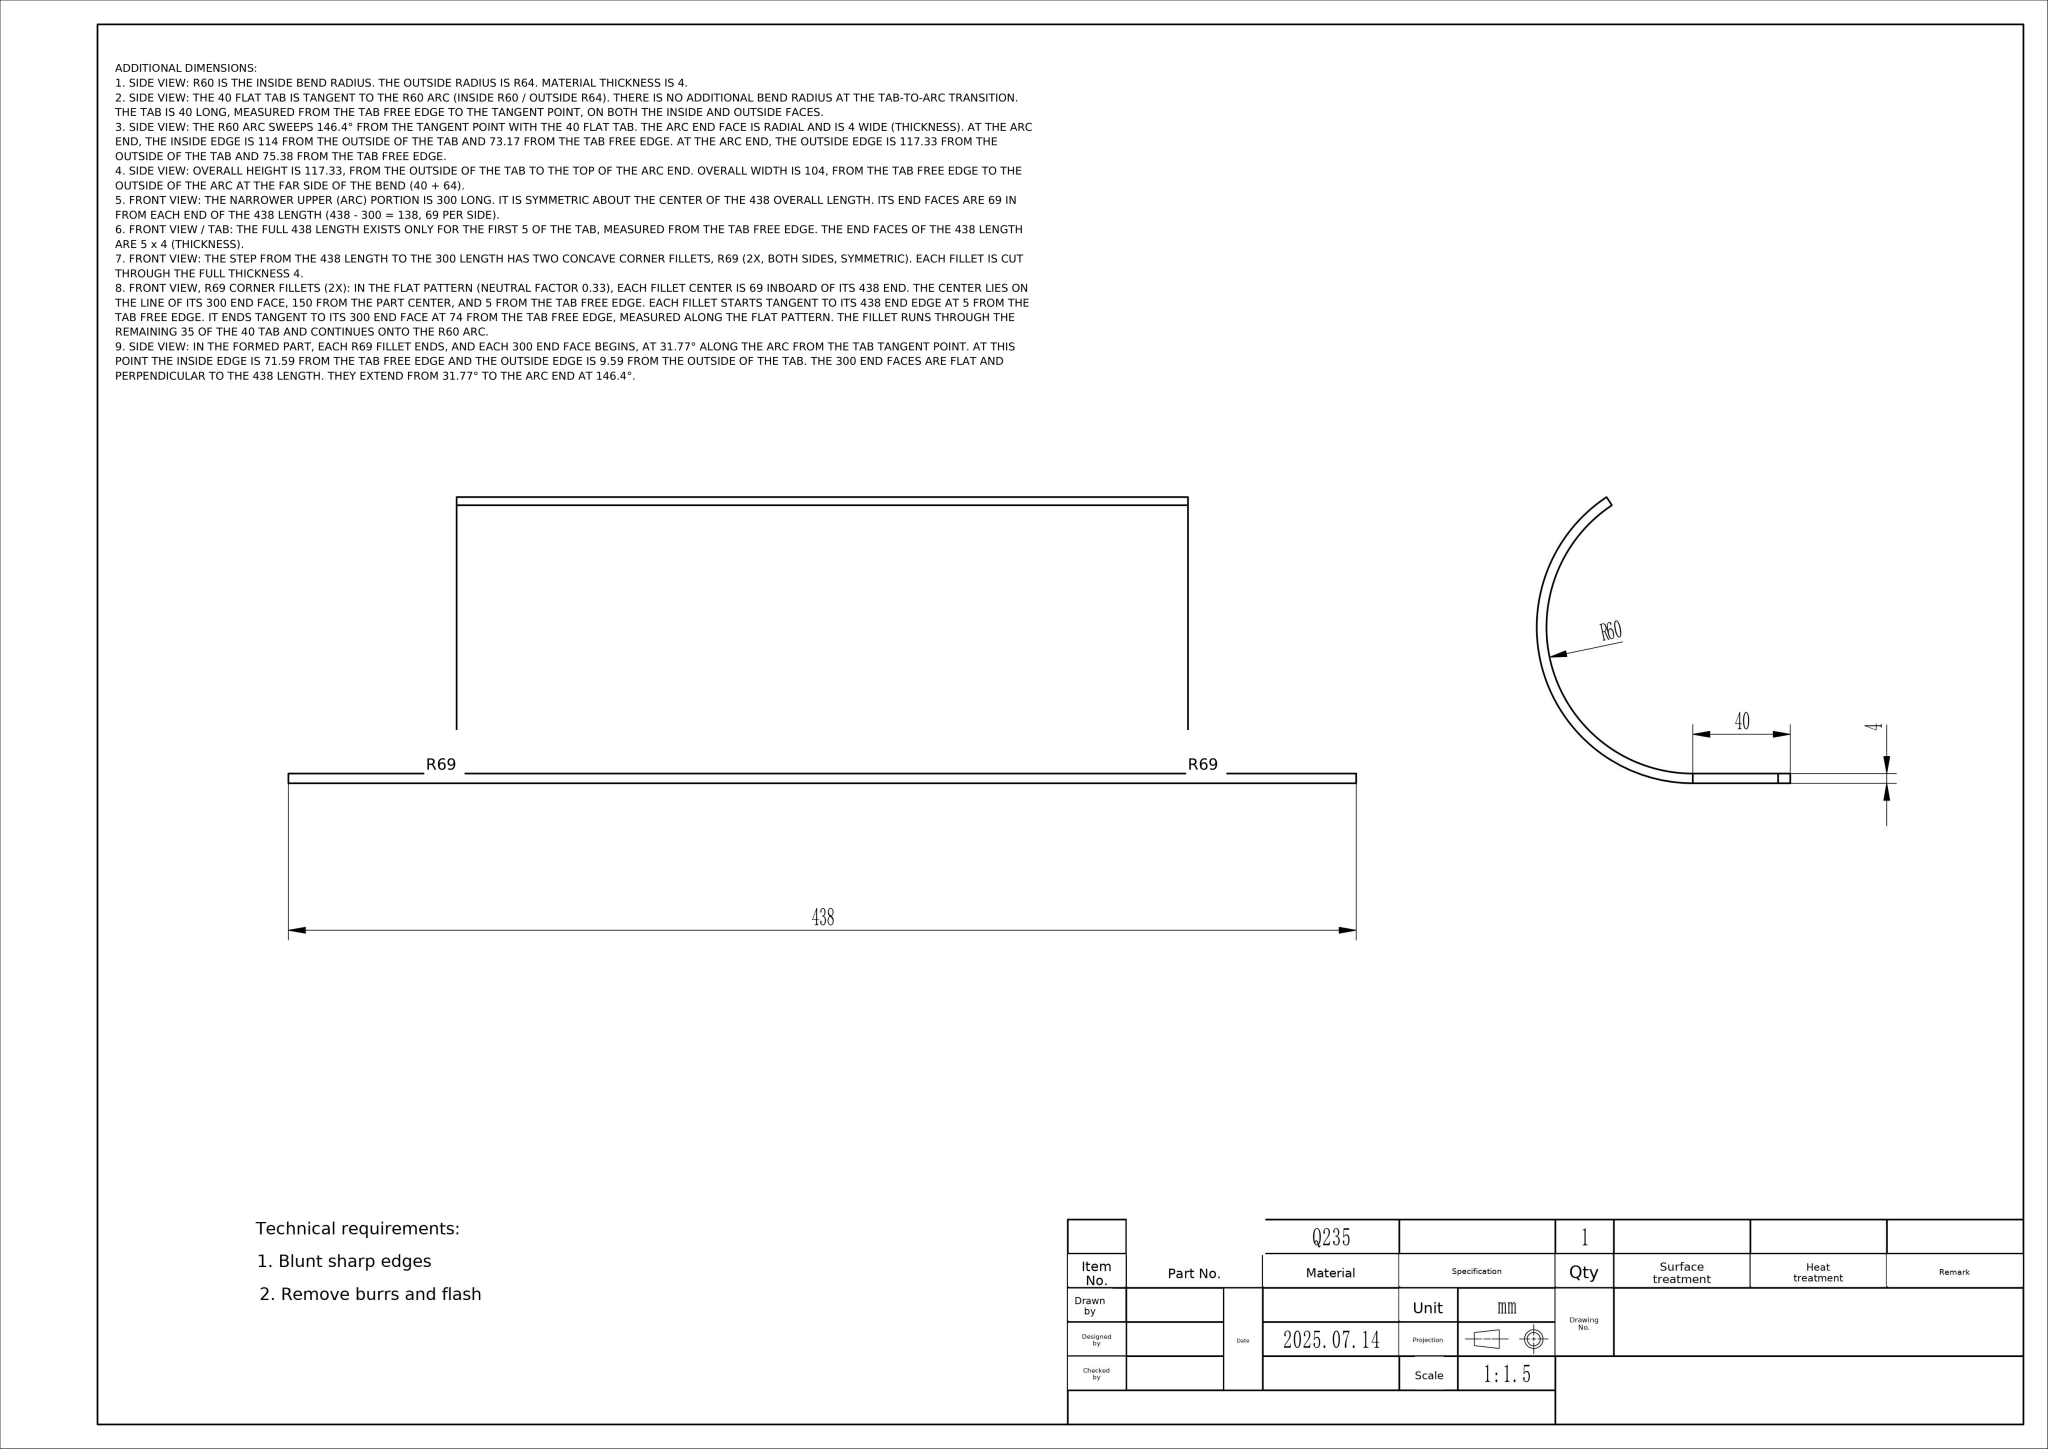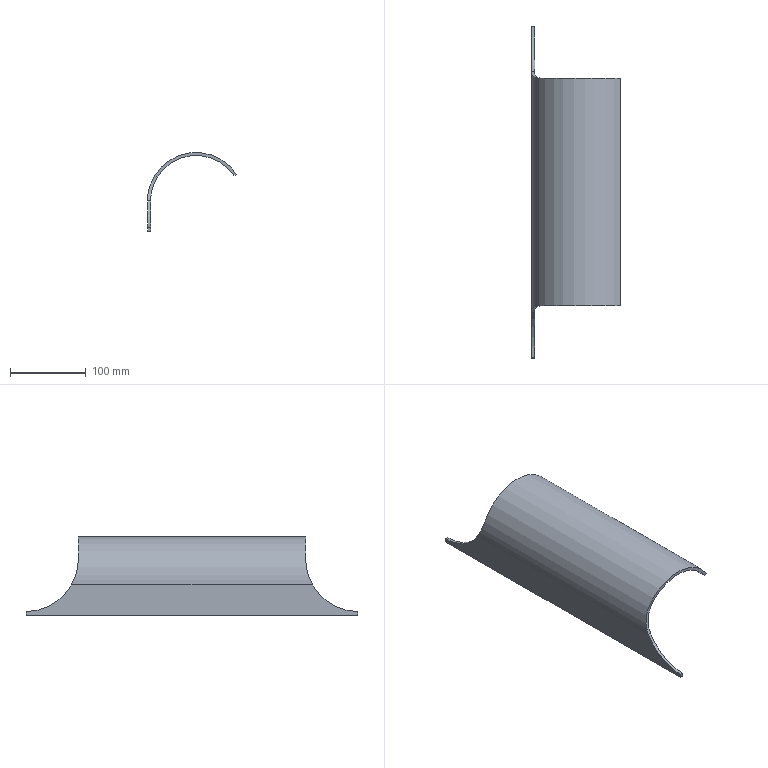Part | NX | mm | 1 solid | 14 faces | box 117.33 x 438 x 104 mm | volume 249102 mm3 | plane 8 | cylinder 4 | spline 2 | commonest cylinder face diameters 138 x2 128 x1 120 x1
STEP:
#1=CARTESIAN_POINT('',(0.,0.,0.));
#2=DIRECTION('',(0.,0.,1.));
#3=DIRECTION('',(1.,0.,0.));
#4=AXIS2_PLACEMENT_3D('',#1,#2,#3);
#5=(LENGTH_UNIT()NAMED_UNIT(*)SI_UNIT(.MILLI.,.METRE.));
#6=UNCERTAINTY_MEASURE_WITH_UNIT(LENGTH_MEASURE(0.0508),#5,'','');
#7=(NAMED_UNIT(*)PLANE_ANGLE_UNIT()SI_UNIT($,.RADIAN.));
#8=PLANE_ANGLE_MEASURE_WITH_UNIT(PLANE_ANGLE_MEASURE(0.01745),#7);
#9=DIMENSIONAL_EXPONENTS(0.,0.,0.,0.,0.,0.,0.);
#10=(CONVERSION_BASED_UNIT('',#8)NAMED_UNIT(#9)PLANE_ANGLE_UNIT());
#11=(NAMED_UNIT(*)SI_UNIT($,.STERADIAN.)SOLID_ANGLE_UNIT());
#12=(GEOMETRIC_REPRESENTATION_CONTEXT(3)GLOBAL_UNCERTAINTY_ASSIGNED_CONTEXT((#6))GLOBAL_UNIT_ASSIGNED_CONTEXT((#5,#10,#11))REPRESENTATION_CONTEXT('',''));
#13=SHAPE_REPRESENTATION('',(#4),#12);
#14=CARTESIAN_POINT('',(-0.,-158.958,40.));
#15=VERTEX_POINT('',#14);
#16=CARTESIAN_POINT('',(0.,-219.,5.));
#17=VERTEX_POINT('',#16);
#18=CARTESIAN_POINT('',(0.,-219.,74.));
#19=DIRECTION('',(-1.,0.,0.));
#20=DIRECTION('',(0.,1.,0.));
#21=AXIS2_PLACEMENT_3D('',#18,#19,#20);
#22=CIRCLE('',#21,69.);
#23=EDGE_CURVE('',#15,#17,#22,.T.);
#24=ORIENTED_EDGE('',*,*,#23,.F.);
#25=CARTESIAN_POINT('',(-4.,-158.958,40.));
#26=VERTEX_POINT('',#25);
#27=CARTESIAN_POINT('',(-4.,-158.958,40.));
#28=DIRECTION('',(-1.,0.,0.));
#29=VECTOR('',#28,1.);
#30=LINE('',#27,#29);
#31=EDGE_CURVE('',#15,#26,#30,.T.);
#32=ORIENTED_EDGE('',*,*,#31,.T.);
#33=CARTESIAN_POINT('',(-4.,-219.,5.));
#34=VERTEX_POINT('',#33);
#35=CARTESIAN_POINT('',(-4.,-219.,74.));
#36=DIRECTION('',(-1.,0.,0.));
#37=DIRECTION('',(0.,1.,0.));
#38=AXIS2_PLACEMENT_3D('',#35,#36,#37);
#39=CIRCLE('',#38,69.);
#40=EDGE_CURVE('',#26,#34,#39,.T.);
#41=ORIENTED_EDGE('',*,*,#40,.T.);
#42=CARTESIAN_POINT('',(-4.,-219.,5.));
#43=DIRECTION('',(-1.,0.,0.));
#44=VECTOR('',#43,1.);
#45=LINE('',#42,#44);
#46=EDGE_CURVE('',#17,#34,#45,.T.);
#47=ORIENTED_EDGE('',*,*,#46,.F.);
#48=EDGE_LOOP('',(#24,#32,#41,#47));
#49=FACE_OUTER_BOUND('',#48,.T.);
#50=CARTESIAN_POINT('',(-4.,-219.,74.));
#51=DIRECTION('',(1.,0.,-0.));
#52=DIRECTION('',(0.,0.,-1.));
#53=AXIS2_PLACEMENT_3D('',#50,#51,#52);
#54=CYLINDRICAL_SURFACE('',#53,69.);
#55=ADVANCED_FACE('',(#49),#54,.F.);
#56=CARTESIAN_POINT('',(0.,219.,0.));
#57=VERTEX_POINT('',#56);
#58=CARTESIAN_POINT('',(0.,-219.,-0.));
#59=VERTEX_POINT('',#58);
#60=CARTESIAN_POINT('',(0.,-150.,0.));
#61=DIRECTION('',(0.,-1.,0.));
#62=VECTOR('',#61,1.);
#63=LINE('',#60,#62);
#64=EDGE_CURVE('',#57,#59,#63,.T.);
#65=ORIENTED_EDGE('',*,*,#64,.T.);
#66=CARTESIAN_POINT('',(-4.,-219.,-0.));
#67=VERTEX_POINT('',#66);
#68=CARTESIAN_POINT('',(-4.,-219.,-0.));
#69=DIRECTION('',(-1.,0.,0.));
#70=VECTOR('',#69,1.);
#71=LINE('',#68,#70);
#72=EDGE_CURVE('',#59,#67,#71,.T.);
#73=ORIENTED_EDGE('',*,*,#72,.T.);
#74=CARTESIAN_POINT('',(-4.,219.,0.));
#75=VERTEX_POINT('',#74);
#76=CARTESIAN_POINT('',(-4.,-150.,0.));
#77=DIRECTION('',(0.,-1.,0.));
#78=VECTOR('',#77,1.);
#79=LINE('',#76,#78);
#80=EDGE_CURVE('',#75,#67,#79,.T.);
#81=ORIENTED_EDGE('',*,*,#80,.F.);
#82=CARTESIAN_POINT('',(-4.,219.,0.));
#83=DIRECTION('',(-1.,0.,0.));
#84=VECTOR('',#83,1.);
#85=LINE('',#82,#84);
#86=EDGE_CURVE('',#57,#75,#85,.T.);
#87=ORIENTED_EDGE('',*,*,#86,.F.);
#88=EDGE_LOOP('',(#65,#73,#81,#87));
#89=FACE_OUTER_BOUND('',#88,.T.);
#90=CARTESIAN_POINT('',(0.,-150.,0.));
#91=DIRECTION('',(0.,0.,1.));
#92=DIRECTION('',(0.,1.,0.));
#93=AXIS2_PLACEMENT_3D('',#90,#91,#92);
#94=PLANE('',#93);
#95=ADVANCED_FACE('',(#89),#94,.F.);
#96=CARTESIAN_POINT('',(-4.,158.958,40.));
#97=VERTEX_POINT('',#96);
#98=CARTESIAN_POINT('',(-4.,-150.,40.));
#99=DIRECTION('',(0.,-1.,0.));
#100=VECTOR('',#99,1.);
#101=LINE('',#98,#100);
#102=EDGE_CURVE('',#97,#26,#101,.T.);
#103=ORIENTED_EDGE('',*,*,#102,.F.);
#104=CARTESIAN_POINT('',(-4.,219.,5.));
#105=VERTEX_POINT('',#104);
#106=CARTESIAN_POINT('',(-4.,219.,74.));
#107=DIRECTION('',(1.,0.,0.));
#108=DIRECTION('',(0.,1.,0.));
#109=AXIS2_PLACEMENT_3D('',#106,#107,#108);
#110=CIRCLE('',#109,69.);
#111=EDGE_CURVE('',#97,#105,#110,.T.);
#112=ORIENTED_EDGE('',*,*,#111,.T.);
#113=CARTESIAN_POINT('',(-4.,219.,0.));
#114=DIRECTION('',(0.,0.,-1.));
#115=VECTOR('',#114,1.);
#116=LINE('',#113,#115);
#117=EDGE_CURVE('',#105,#75,#116,.T.);
#118=ORIENTED_EDGE('',*,*,#117,.T.);
#119=ORIENTED_EDGE('',*,*,#80,.T.);
#120=CARTESIAN_POINT('',(-4.,-219.,-0.));
#121=DIRECTION('',(0.,0.,-1.));
#122=VECTOR('',#121,1.);
#123=LINE('',#120,#122);
#124=EDGE_CURVE('',#34,#67,#123,.T.);
#125=ORIENTED_EDGE('',*,*,#124,.F.);
#126=ORIENTED_EDGE('',*,*,#40,.F.);
#127=EDGE_LOOP('',(#103,#112,#118,#119,#125,#126));
#128=FACE_OUTER_BOUND('',#127,.T.);
#129=CARTESIAN_POINT('',(-4.,-150.,0.));
#130=DIRECTION('',(-1.,0.,0.));
#131=DIRECTION('',(0.,0.,1.));
#132=AXIS2_PLACEMENT_3D('',#129,#130,#131);
#133=PLANE('',#132);
#134=ADVANCED_FACE('',(#128),#133,.T.);
#135=ORIENTED_EDGE('',*,*,#64,.F.);
#136=CARTESIAN_POINT('',(0.,219.,5.));
#137=VERTEX_POINT('',#136);
#138=CARTESIAN_POINT('',(0.,219.,0.));
#139=DIRECTION('',(0.,0.,-1.));
#140=VECTOR('',#139,1.);
#141=LINE('',#138,#140);
#142=EDGE_CURVE('',#137,#57,#141,.T.);
#143=ORIENTED_EDGE('',*,*,#142,.F.);
#144=CARTESIAN_POINT('',(0.,158.958,40.));
#145=VERTEX_POINT('',#144);
#146=CARTESIAN_POINT('',(0.,219.,74.));
#147=DIRECTION('',(1.,0.,0.));
#148=DIRECTION('',(0.,1.,0.));
#149=AXIS2_PLACEMENT_3D('',#146,#147,#148);
#150=CIRCLE('',#149,69.);
#151=EDGE_CURVE('',#145,#137,#150,.T.);
#152=ORIENTED_EDGE('',*,*,#151,.F.);
#153=CARTESIAN_POINT('',(0.,-150.,40.));
#154=DIRECTION('',(0.,-1.,0.));
#155=VECTOR('',#154,1.);
#156=LINE('',#153,#155);
#157=EDGE_CURVE('',#145,#15,#156,.T.);
#158=ORIENTED_EDGE('',*,*,#157,.T.);
#159=ORIENTED_EDGE('',*,*,#23,.T.);
#160=CARTESIAN_POINT('',(0.,-219.,-0.));
#161=DIRECTION('',(0.,0.,-1.));
#162=VECTOR('',#161,1.);
#163=LINE('',#160,#162);
#164=EDGE_CURVE('',#17,#59,#163,.T.);
#165=ORIENTED_EDGE('',*,*,#164,.T.);
#166=EDGE_LOOP('',(#135,#143,#152,#158,#159,#165));
#167=FACE_OUTER_BOUND('',#166,.T.);
#168=CARTESIAN_POINT('',(0.,-150.,0.));
#169=DIRECTION('',(-1.,0.,0.));
#170=DIRECTION('',(0.,0.,1.));
#171=AXIS2_PLACEMENT_3D('',#168,#169,#170);
#172=PLANE('',#171);
#173=ADVANCED_FACE('',(#167),#172,.F.);
#174=ORIENTED_EDGE('',*,*,#142,.T.);
#175=ORIENTED_EDGE('',*,*,#86,.T.);
#176=ORIENTED_EDGE('',*,*,#117,.F.);
#177=CARTESIAN_POINT('',(-4.,219.,5.));
#178=DIRECTION('',(-1.,0.,0.));
#179=VECTOR('',#178,1.);
#180=LINE('',#177,#179);
#181=EDGE_CURVE('',#137,#105,#180,.T.);
#182=ORIENTED_EDGE('',*,*,#181,.F.);
#183=EDGE_LOOP('',(#174,#175,#176,#182));
#184=FACE_OUTER_BOUND('',#183,.T.);
#185=CARTESIAN_POINT('',(-4.,219.,0.));
#186=DIRECTION('',(0.,1.,0.));
#187=DIRECTION('',(0.,0.,1.));
#188=AXIS2_PLACEMENT_3D('',#185,#186,#187);
#189=PLANE('',#188);
#190=ADVANCED_FACE('',(#184),#189,.T.);
#191=CARTESIAN_POINT('',(-4.,158.958,40.));
#192=DIRECTION('',(-1.,0.,0.));
#193=VECTOR('',#192,1.);
#194=LINE('',#191,#193);
#195=EDGE_CURVE('',#145,#97,#194,.T.);
#196=ORIENTED_EDGE('',*,*,#195,.F.);
#197=ORIENTED_EDGE('',*,*,#151,.T.);
#198=ORIENTED_EDGE('',*,*,#181,.T.);
#199=ORIENTED_EDGE('',*,*,#111,.F.);
#200=EDGE_LOOP('',(#196,#197,#198,#199));
#201=FACE_OUTER_BOUND('',#200,.T.);
#202=CARTESIAN_POINT('',(-4.,219.,74.));
#203=DIRECTION('',(1.,0.,-0.));
#204=DIRECTION('',(0.,0.,-1.));
#205=AXIS2_PLACEMENT_3D('',#202,#203,#204);
#206=CYLINDRICAL_SURFACE('',#205,69.);
#207=ADVANCED_FACE('',(#201),#206,.F.);
#208=ORIENTED_EDGE('',*,*,#164,.F.);
#209=ORIENTED_EDGE('',*,*,#46,.T.);
#210=ORIENTED_EDGE('',*,*,#124,.T.);
#211=ORIENTED_EDGE('',*,*,#72,.F.);
#212=EDGE_LOOP('',(#208,#209,#210,#211));
#213=FACE_OUTER_BOUND('',#212,.T.);
#214=CARTESIAN_POINT('',(-4.,-219.,-0.));
#215=DIRECTION('',(0.,1.,0.));
#216=DIRECTION('',(0.,0.,1.));
#217=AXIS2_PLACEMENT_3D('',#214,#215,#216);
#218=PLANE('',#217);
#219=ADVANCED_FACE('',(#213),#218,.F.);
#220=CARTESIAN_POINT('',(110.,150.,73.166));
#221=VERTEX_POINT('',#220);
#222=CARTESIAN_POINT('',(113.333,150.,75.377));
#223=VERTEX_POINT('',#222);
#224=CARTESIAN_POINT('',(113.333,150.,75.377));
#225=DIRECTION('',(0.8333,0.,0.5528));
#226=VECTOR('',#225,1.);
#227=LINE('',#224,#226);
#228=EDGE_CURVE('',#221,#223,#227,.T.);
#229=ORIENTED_EDGE('',*,*,#228,.F.);
#230=CARTESIAN_POINT('',(8.989,150.,71.589));
#231=VERTEX_POINT('',#230);
#232=CARTESIAN_POINT('',(60.,150.,40.));
#233=DIRECTION('',(-0.,-1.,-0.));
#234=DIRECTION('',(0.,0.,1.));
#235=AXIS2_PLACEMENT_3D('',#232,#233,#234);
#236=CIRCLE('',#235,60.);
#237=EDGE_CURVE('',#221,#231,#236,.T.);
#238=ORIENTED_EDGE('',*,*,#237,.T.);
#239=CARTESIAN_POINT('',(5.588,150.,73.695));
#240=VERTEX_POINT('',#239);
#241=CARTESIAN_POINT('',(8.989,150.,71.589));
#242=DIRECTION('',(0.8502,0.,-0.5265));
#243=VECTOR('',#242,1.);
#244=LINE('',#241,#243);
#245=EDGE_CURVE('',#240,#231,#244,.T.);
#246=ORIENTED_EDGE('',*,*,#245,.F.);
#247=CARTESIAN_POINT('',(60.,150.,40.));
#248=DIRECTION('',(-0.,-1.,-0.));
#249=DIRECTION('',(1.,0.,0.));
#250=AXIS2_PLACEMENT_3D('',#247,#248,#249);
#251=CIRCLE('',#250,64.);
#252=EDGE_CURVE('',#223,#240,#251,.T.);
#253=ORIENTED_EDGE('',*,*,#252,.F.);
#254=EDGE_LOOP('',(#229,#238,#246,#253));
#255=FACE_OUTER_BOUND('',#254,.T.);
#256=CARTESIAN_POINT('',(60.,150.,40.));
#257=DIRECTION('',(0.,1.,0.));
#258=DIRECTION('',(0.,-0.,1.));
#259=AXIS2_PLACEMENT_3D('',#256,#257,#258);
#260=PLANE('',#259);
#261=ADVANCED_FACE('',(#255),#260,.T.);
#262=ORIENTED_EDGE('',*,*,#245,.T.);
#263=CARTESIAN_POINT('',(8.989,150.,71.589));
#264=CARTESIAN_POINT('',(7.463,150.,69.125));
#265=CARTESIAN_POINT('',(6.117,150.191,66.549));
#266=CARTESIAN_POINT('',(3.825,150.952,61.276));
#267=CARTESIAN_POINT('',(2.88,151.522,58.578));
#268=CARTESIAN_POINT('',(1.397,153.032,53.172));
#269=CARTESIAN_POINT('',(0.8583,153.972,50.463));
#270=CARTESIAN_POINT('',(0.1601,156.205,45.138));
#271=CARTESIAN_POINT('',(0.,157.499,42.522));
#272=CARTESIAN_POINT('',(0.,158.958,40.));
#273=B_SPLINE_CURVE_WITH_KNOTS('',3,(#263,#264,#265,#266,#267,#268,#269,#270,#271,#272),.UNSPECIFIED.,.F.,.F.,(4,2,2,2,4),(0.,0.25,0.5,0.75,1.),.UNSPECIFIED.);
#274=EDGE_CURVE('',#231,#145,#273,.T.);
#275=ORIENTED_EDGE('',*,*,#274,.T.);
#276=ORIENTED_EDGE('',*,*,#195,.T.);
#277=CARTESIAN_POINT('',(5.588,150.,73.695));
#278=CARTESIAN_POINT('',(2.332,150.,68.438));
#279=CARTESIAN_POINT('',(-0.1369,150.767,62.701));
#280=CARTESIAN_POINT('',(-3.301,153.787,51.166));
#281=CARTESIAN_POINT('',(-4.,156.039,45.381));
#282=CARTESIAN_POINT('',(-4.,158.958,40.));
#283=B_SPLINE_CURVE_WITH_KNOTS('',3,(#277,#278,#279,#280,#281,#282),.UNSPECIFIED.,.F.,.F.,(4,2,4),(0.,0.5,1.),.UNSPECIFIED.);
#284=EDGE_CURVE('',#240,#97,#283,.T.);
#285=ORIENTED_EDGE('',*,*,#284,.F.);
#286=EDGE_LOOP('',(#262,#275,#276,#285));
#287=FACE_OUTER_BOUND('',#286,.T.);
#288=CARTESIAN_POINT('',(-4.,158.958,40.));
#289=CARTESIAN_POINT('',(-4.,157.499,42.691));
#290=CARTESIAN_POINT('',(-3.829,156.205,45.48));
#291=CARTESIAN_POINT('',(-3.085,153.972,51.16));
#292=CARTESIAN_POINT('',(-2.51,153.032,54.05));
#293=CARTESIAN_POINT('',(-0.9281,151.522,59.817));
#294=CARTESIAN_POINT('',(0.08016,150.952,62.694));
#295=CARTESIAN_POINT('',(2.524,150.191,68.319));
#296=CARTESIAN_POINT('',(3.96,150.,71.066));
#297=CARTESIAN_POINT('',(5.588,150.,73.695));
#298=CARTESIAN_POINT('',(0.,158.958,40.));
#299=CARTESIAN_POINT('',(0.,157.499,42.522));
#300=CARTESIAN_POINT('',(0.1601,156.205,45.138));
#301=CARTESIAN_POINT('',(0.8583,153.972,50.463));
#302=CARTESIAN_POINT('',(1.397,153.032,53.172));
#303=CARTESIAN_POINT('',(2.88,151.522,58.578));
#304=CARTESIAN_POINT('',(3.825,150.952,61.276));
#305=CARTESIAN_POINT('',(6.117,150.191,66.549));
#306=CARTESIAN_POINT('',(7.463,150.,69.125));
#307=CARTESIAN_POINT('',(8.989,150.,71.589));
#308=B_SPLINE_SURFACE_WITH_KNOTS('',1,3,((#288,#289,#290,#291,#292,#293,#294,#295,#296,#297),(#298,#299,#300,#301,#302,#303,#304,#305,#306,#307)),.UNSPECIFIED.,.F.,.F.,.F.,(2,2),(4,2,2,2,4),(0.,1.),(0.,0.25,0.5,0.75,1.),.UNSPECIFIED.);
#309=ADVANCED_FACE('',(#287),#308,.F.);
#310=ORIENTED_EDGE('',*,*,#31,.F.);
#311=CARTESIAN_POINT('',(8.989,-150.,71.589));
#312=VERTEX_POINT('',#311);
#313=CARTESIAN_POINT('',(8.989,-150.,71.589));
#314=CARTESIAN_POINT('',(5.937,-150.,66.66));
#315=CARTESIAN_POINT('',(3.622,-150.767,61.282));
#316=CARTESIAN_POINT('',(0.6549,-153.787,50.468));
#317=CARTESIAN_POINT('',(0.,-156.039,45.045));
#318=CARTESIAN_POINT('',(0.,-158.958,40.));
#319=B_SPLINE_CURVE_WITH_KNOTS('',3,(#313,#314,#315,#316,#317,#318),.UNSPECIFIED.,.F.,.F.,(4,2,4),(0.,0.5,1.),.UNSPECIFIED.);
#320=EDGE_CURVE('',#312,#15,#319,.T.);
#321=ORIENTED_EDGE('',*,*,#320,.F.);
#322=CARTESIAN_POINT('',(5.588,-150.,73.695));
#323=VERTEX_POINT('',#322);
#324=CARTESIAN_POINT('',(5.588,-150.,73.695));
#325=DIRECTION('',(-0.8502,0.,0.5265));
#326=VECTOR('',#325,1.);
#327=LINE('',#324,#326);
#328=EDGE_CURVE('',#312,#323,#327,.T.);
#329=ORIENTED_EDGE('',*,*,#328,.T.);
#330=CARTESIAN_POINT('',(5.588,-150.,73.695));
#331=CARTESIAN_POINT('',(3.96,-150.,71.066));
#332=CARTESIAN_POINT('',(2.524,-150.191,68.319));
#333=CARTESIAN_POINT('',(0.08016,-150.952,62.694));
#334=CARTESIAN_POINT('',(-0.9281,-151.522,59.817));
#335=CARTESIAN_POINT('',(-2.51,-153.032,54.05));
#336=CARTESIAN_POINT('',(-3.085,-153.972,51.16));
#337=CARTESIAN_POINT('',(-3.829,-156.205,45.48));
#338=CARTESIAN_POINT('',(-4.,-157.499,42.691));
#339=CARTESIAN_POINT('',(-4.,-158.958,40.));
#340=B_SPLINE_CURVE_WITH_KNOTS('',3,(#330,#331,#332,#333,#334,#335,#336,#337,#338,#339),.UNSPECIFIED.,.F.,.F.,(4,2,2,2,4),(0.,0.25,0.5,0.75,1.),.UNSPECIFIED.);
#341=EDGE_CURVE('',#323,#26,#340,.T.);
#342=ORIENTED_EDGE('',*,*,#341,.T.);
#343=EDGE_LOOP('',(#310,#321,#329,#342));
#344=FACE_OUTER_BOUND('',#343,.T.);
#345=CARTESIAN_POINT('',(-4.,-158.958,40.));
#346=CARTESIAN_POINT('',(-4.,-157.499,42.691));
#347=CARTESIAN_POINT('',(-3.829,-156.205,45.48));
#348=CARTESIAN_POINT('',(-3.085,-153.972,51.16));
#349=CARTESIAN_POINT('',(-2.51,-153.032,54.05));
#350=CARTESIAN_POINT('',(-0.9281,-151.522,59.817));
#351=CARTESIAN_POINT('',(0.08016,-150.952,62.694));
#352=CARTESIAN_POINT('',(2.524,-150.191,68.319));
#353=CARTESIAN_POINT('',(3.96,-150.,71.066));
#354=CARTESIAN_POINT('',(5.588,-150.,73.695));
#355=CARTESIAN_POINT('',(0.,-158.958,40.));
#356=CARTESIAN_POINT('',(0.,-157.499,42.522));
#357=CARTESIAN_POINT('',(0.1601,-156.205,45.138));
#358=CARTESIAN_POINT('',(0.8583,-153.972,50.463));
#359=CARTESIAN_POINT('',(1.397,-153.032,53.172));
#360=CARTESIAN_POINT('',(2.88,-151.522,58.578));
#361=CARTESIAN_POINT('',(3.825,-150.952,61.276));
#362=CARTESIAN_POINT('',(6.117,-150.191,66.549));
#363=CARTESIAN_POINT('',(7.463,-150.,69.125));
#364=CARTESIAN_POINT('',(8.989,-150.,71.589));
#365=B_SPLINE_SURFACE_WITH_KNOTS('',1,3,((#345,#346,#347,#348,#349,#350,#351,#352,#353,#354),(#355,#356,#357,#358,#359,#360,#361,#362,#363,#364)),.UNSPECIFIED.,.F.,.F.,.F.,(2,2),(4,2,2,2,4),(0.,1.),(0.,0.25,0.5,0.75,1.),.UNSPECIFIED.);
#366=ADVANCED_FACE('',(#344),#365,.T.);
#367=ORIENTED_EDGE('',*,*,#328,.F.);
#368=CARTESIAN_POINT('',(110.,-150.,73.166));
#369=VERTEX_POINT('',#368);
#370=CARTESIAN_POINT('',(60.,-150.,40.));
#371=DIRECTION('',(-0.,-1.,-0.));
#372=DIRECTION('',(0.,0.,1.));
#373=AXIS2_PLACEMENT_3D('',#370,#371,#372);
#374=CIRCLE('',#373,60.);
#375=EDGE_CURVE('',#369,#312,#374,.T.);
#376=ORIENTED_EDGE('',*,*,#375,.F.);
#377=CARTESIAN_POINT('',(113.333,-150.,75.377));
#378=VERTEX_POINT('',#377);
#379=CARTESIAN_POINT('',(113.333,-150.,75.377));
#380=DIRECTION('',(0.8333,-0.,0.5528));
#381=VECTOR('',#380,1.);
#382=LINE('',#379,#381);
#383=EDGE_CURVE('',#369,#378,#382,.T.);
#384=ORIENTED_EDGE('',*,*,#383,.T.);
#385=CARTESIAN_POINT('',(60.,-150.,40.));
#386=DIRECTION('',(-0.,-1.,-0.));
#387=DIRECTION('',(1.,0.,0.));
#388=AXIS2_PLACEMENT_3D('',#385,#386,#387);
#389=CIRCLE('',#388,64.);
#390=EDGE_CURVE('',#378,#323,#389,.T.);
#391=ORIENTED_EDGE('',*,*,#390,.T.);
#392=EDGE_LOOP('',(#367,#376,#384,#391));
#393=FACE_OUTER_BOUND('',#392,.T.);
#394=CARTESIAN_POINT('',(60.,-150.,40.));
#395=DIRECTION('',(0.,1.,0.));
#396=DIRECTION('',(0.,-0.,1.));
#397=AXIS2_PLACEMENT_3D('',#394,#395,#396);
#398=PLANE('',#397);
#399=ADVANCED_FACE('',(#393),#398,.F.);
#400=CARTESIAN_POINT('',(110.,-158.958,73.166));
#401=DIRECTION('',(-0.,-1.,-0.));
#402=VECTOR('',#401,1.);
#403=LINE('',#400,#402);
#404=EDGE_CURVE('',#221,#369,#403,.T.);
#405=ORIENTED_EDGE('',*,*,#404,.F.);
#406=ORIENTED_EDGE('',*,*,#228,.T.);
#407=CARTESIAN_POINT('',(113.333,150.,75.377));
#408=DIRECTION('',(-0.,-1.,0.));
#409=VECTOR('',#408,1.);
#410=LINE('',#407,#409);
#411=EDGE_CURVE('',#223,#378,#410,.T.);
#412=ORIENTED_EDGE('',*,*,#411,.T.);
#413=ORIENTED_EDGE('',*,*,#383,.F.);
#414=EDGE_LOOP('',(#405,#406,#412,#413));
#415=FACE_OUTER_BOUND('',#414,.T.);
#416=CARTESIAN_POINT('',(113.333,0.,75.377));
#417=DIRECTION('',(-0.5528,0.,0.8333));
#418=DIRECTION('',(-0.,-1.,0.));
#419=AXIS2_PLACEMENT_3D('',#416,#417,#418);
#420=PLANE('',#419);
#421=ADVANCED_FACE('',(#415),#420,.F.);
#422=ORIENTED_EDGE('',*,*,#390,.F.);
#423=ORIENTED_EDGE('',*,*,#411,.F.);
#424=ORIENTED_EDGE('',*,*,#252,.T.);
#425=ORIENTED_EDGE('',*,*,#284,.T.);
#426=ORIENTED_EDGE('',*,*,#102,.T.);
#427=ORIENTED_EDGE('',*,*,#341,.F.);
#428=EDGE_LOOP('',(#422,#423,#424,#425,#426,#427));
#429=FACE_OUTER_BOUND('',#428,.T.);
#430=CARTESIAN_POINT('',(60.,-158.958,40.));
#431=DIRECTION('',(0.,1.,0.));
#432=DIRECTION('',(1.,0.,0.));
#433=AXIS2_PLACEMENT_3D('',#430,#431,#432);
#434=CYLINDRICAL_SURFACE('',#433,64.);
#435=ADVANCED_FACE('',(#429),#434,.T.);
#436=ORIENTED_EDGE('',*,*,#375,.T.);
#437=ORIENTED_EDGE('',*,*,#320,.T.);
#438=ORIENTED_EDGE('',*,*,#157,.F.);
#439=ORIENTED_EDGE('',*,*,#274,.F.);
#440=ORIENTED_EDGE('',*,*,#237,.F.);
#441=ORIENTED_EDGE('',*,*,#404,.T.);
#442=EDGE_LOOP('',(#436,#437,#438,#439,#440,#441));
#443=FACE_OUTER_BOUND('',#442,.T.);
#444=CARTESIAN_POINT('',(60.,-158.958,40.));
#445=DIRECTION('',(0.,1.,0.));
#446=DIRECTION('',(1.,0.,0.));
#447=AXIS2_PLACEMENT_3D('',#444,#445,#446);
#448=CYLINDRICAL_SURFACE('',#447,60.);
#449=ADVANCED_FACE('',(#443),#448,.F.);
#450=CLOSED_SHELL('',(#55,#95,#134,#173,#190,#207,#219,#261,#309,#366,#399,#421,#435,#449));
#451=MANIFOLD_SOLID_BREP('',#450);
#452=ADVANCED_BREP_SHAPE_REPRESENTATION('',(#451),#12);
#453=SHAPE_REPRESENTATION_RELATIONSHIP('','',#13,#452);
#454=PRESENTATION_LAYER_ASSIGNMENT('','',(#451));
#455=COLOUR_RGB('',0.5961,0.6667,0.6863);
#456=FILL_AREA_STYLE_COLOUR('',#455);
#457=FILL_AREA_STYLE('',(#456));
#458=SURFACE_STYLE_FILL_AREA(#457);
#459=SURFACE_SIDE_STYLE('',(#458));
#460=SURFACE_STYLE_USAGE(.BOTH.,#459);
#461=PRESENTATION_STYLE_ASSIGNMENT((#460));
#462=STYLED_ITEM('',(#461),#451);
#463=MECHANICAL_DESIGN_GEOMETRIC_PRESENTATION_REPRESENTATION('',(#462),#12);